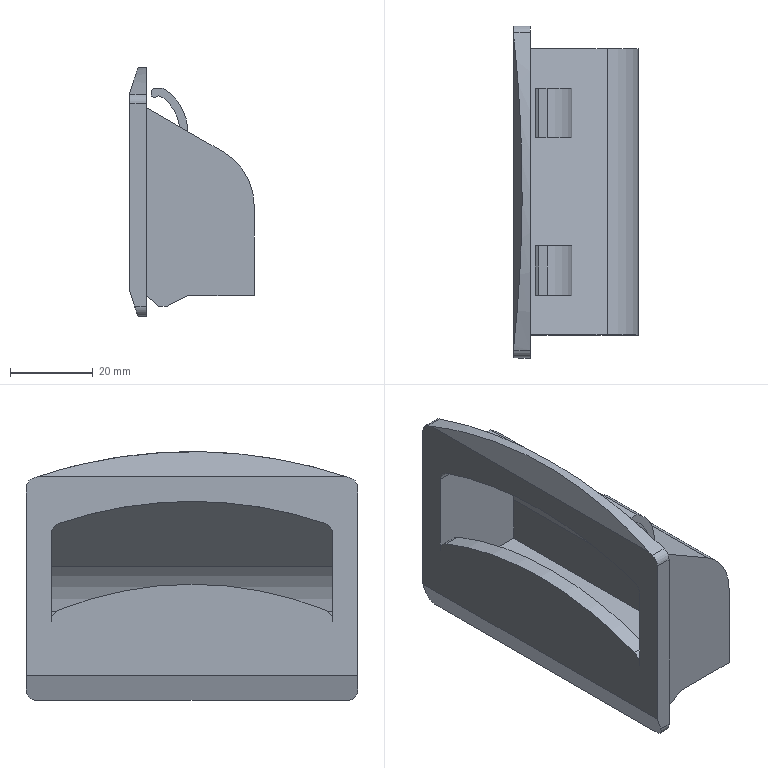Component | SolidWorks | DoorHandleUWAUNJ80-2-1 | 1 solid | 57 faces | volume 41505 mm3 | plane 40 | cylinder 17 | commonest cylinder face diameters 6 x4 5 x4 30 x2 20 x2 24 x2 172.143 x1 198.667 x1 235.571 x1